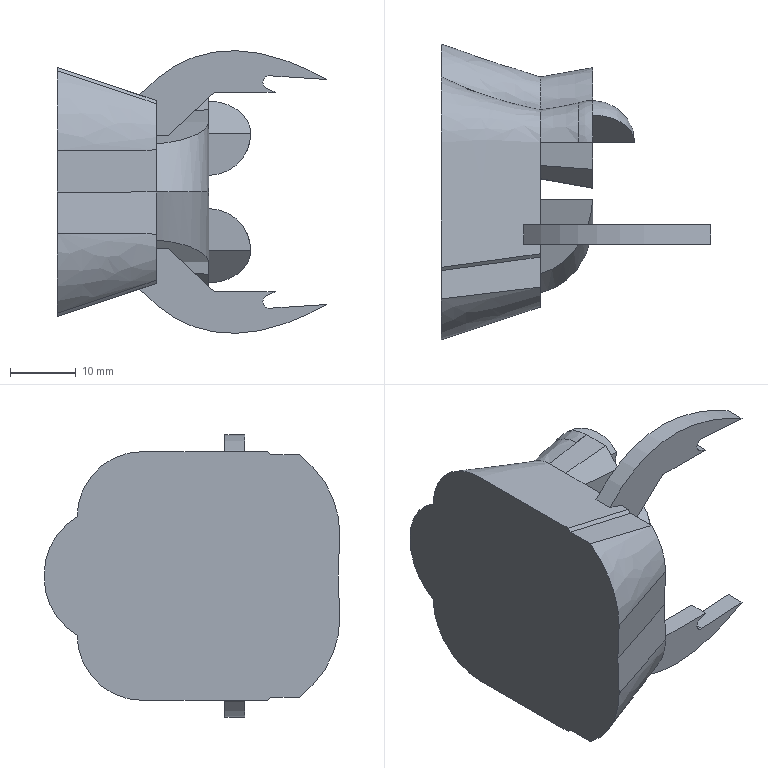Component | SolidWorks | Part13-1 | 1 solid | 58 faces | volume 22847 mm3 | plane 38 | spline 7 | cone 5 | sphere 4 | cylinder 4 | commonest cylinder face diameters 2 x2 20 x2